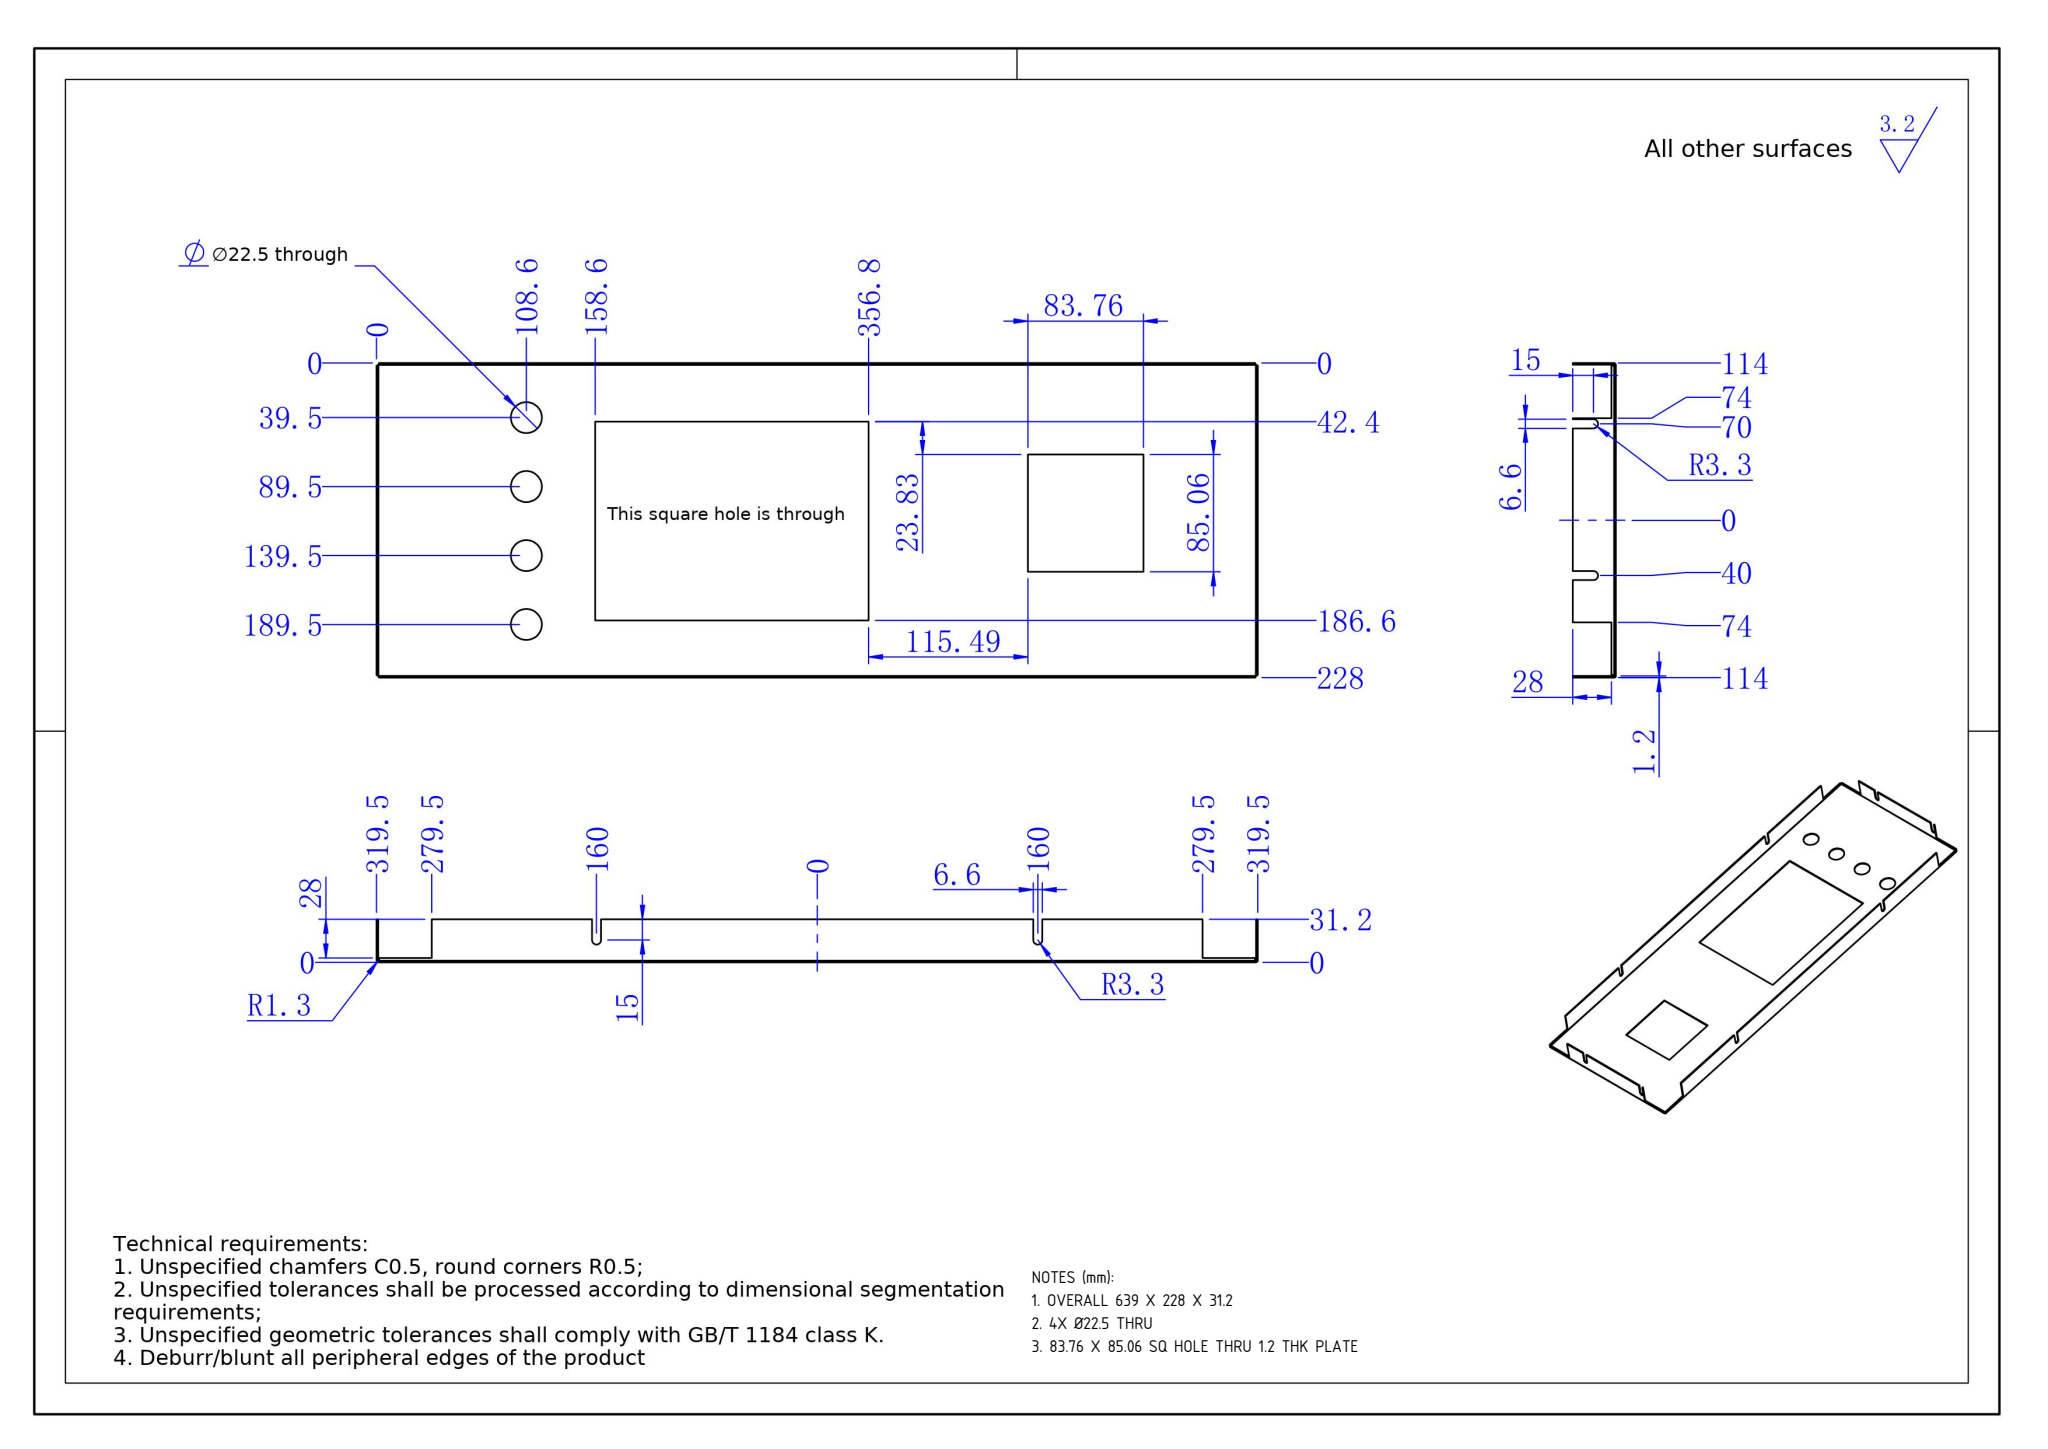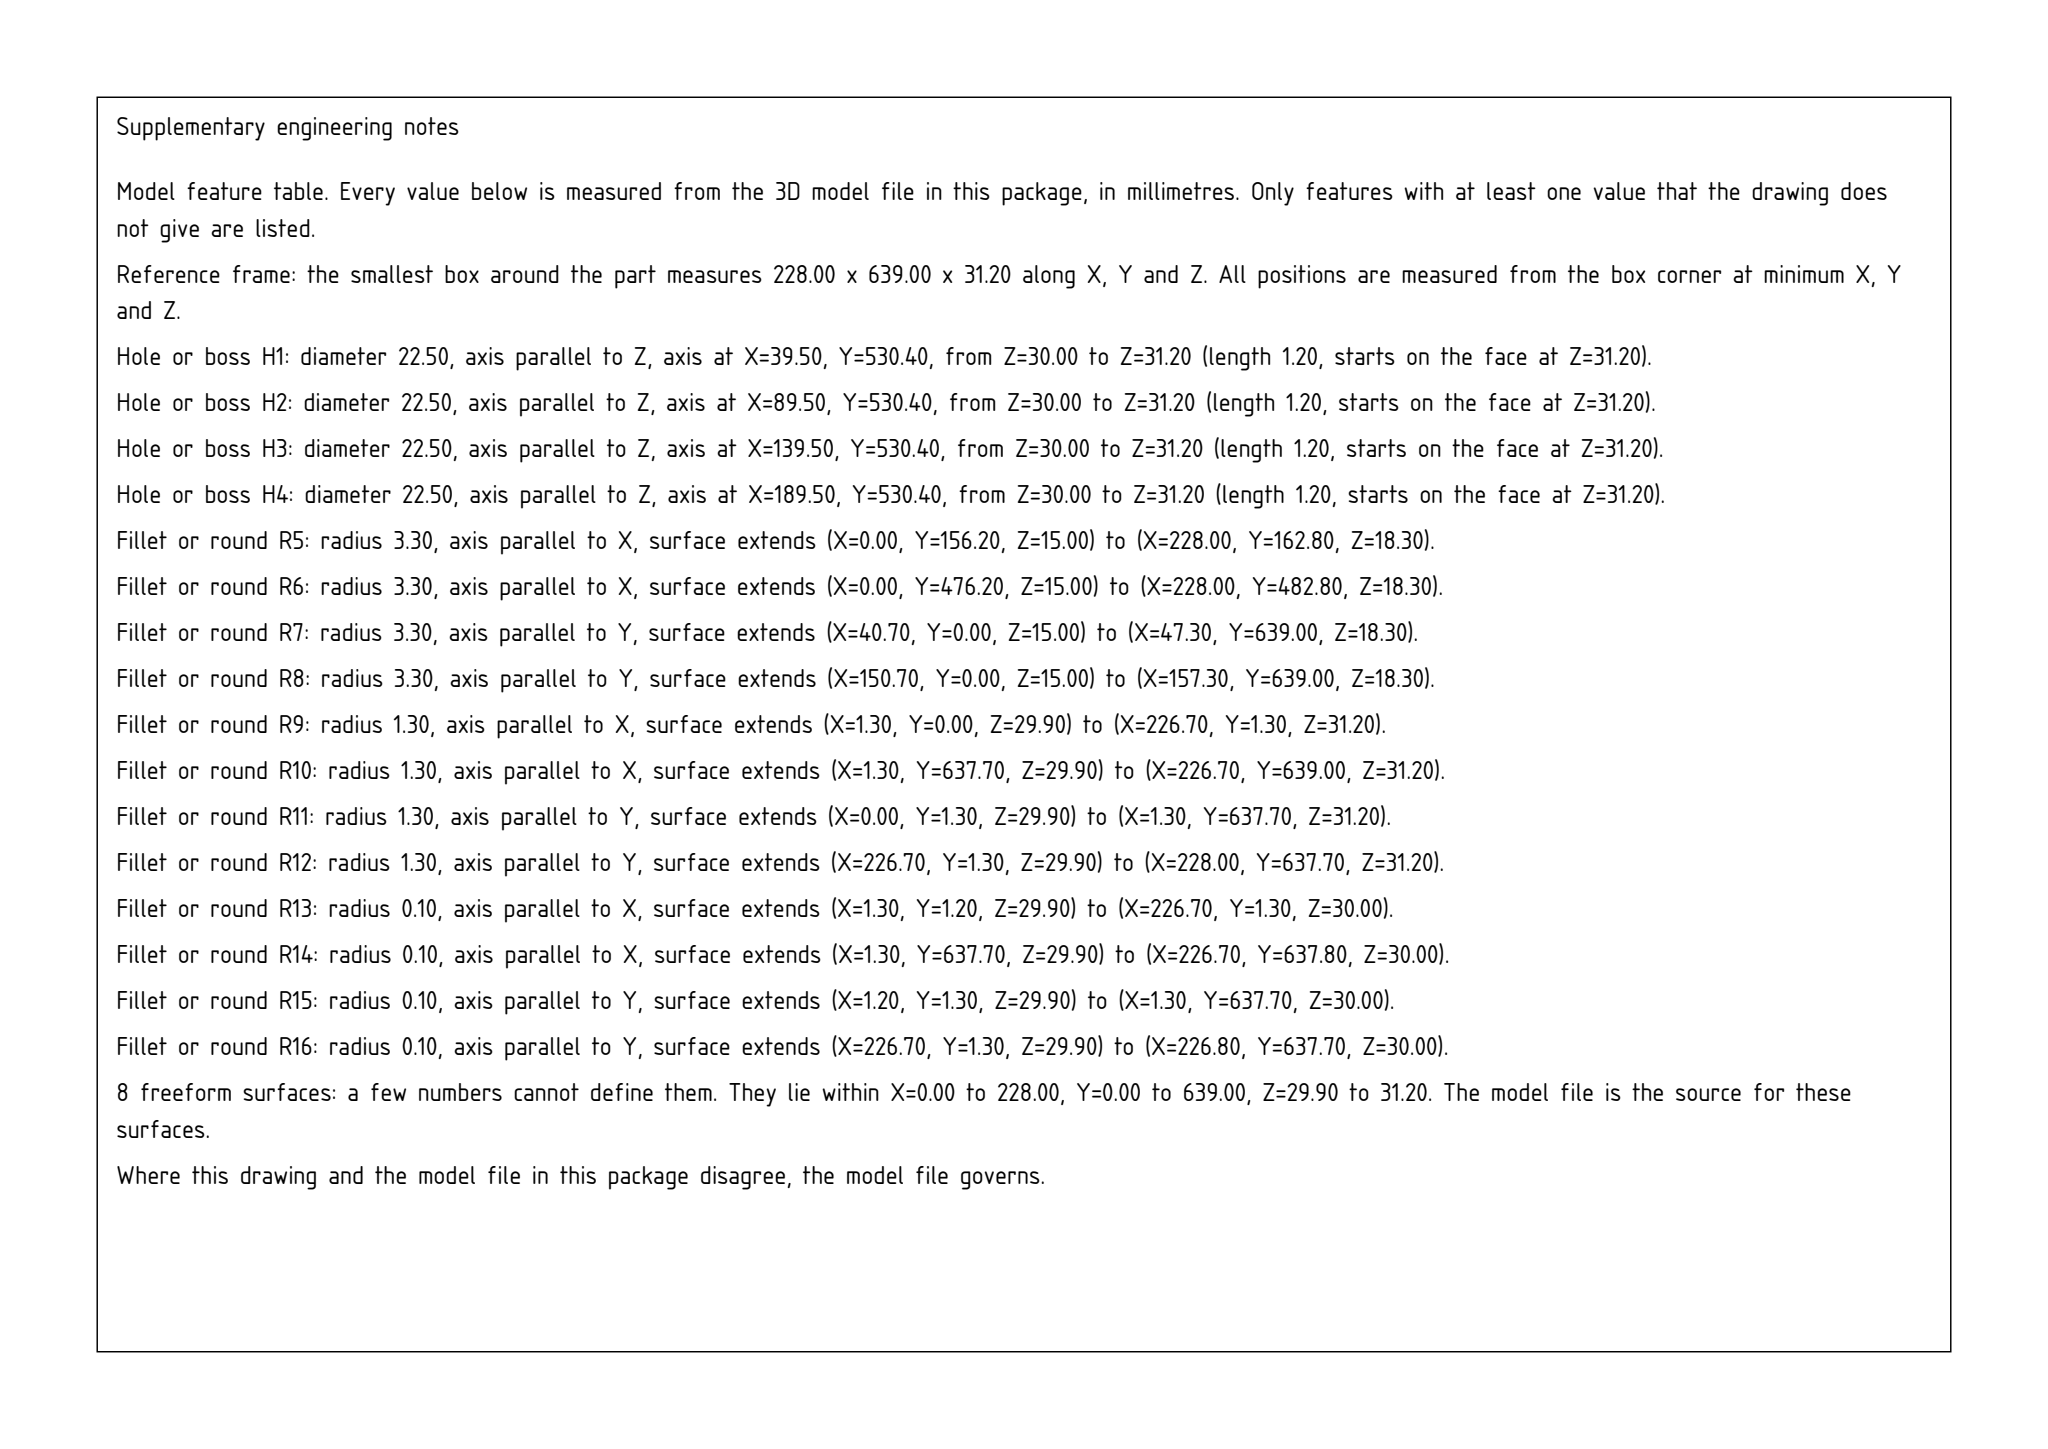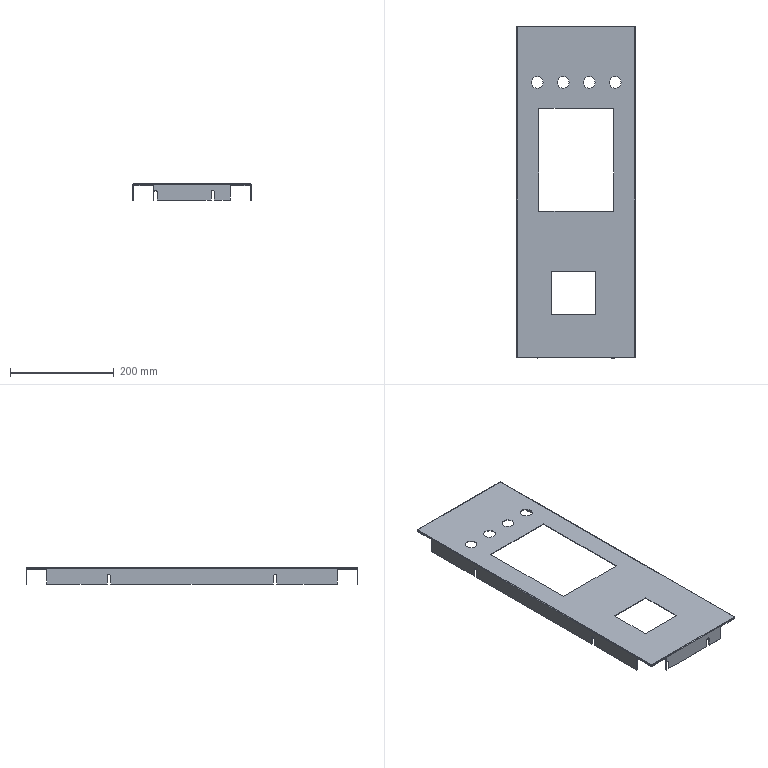Part | SolidWorks | mm | 1 solid | 106 faces | box 228 x 639 x 31.2 mm | volume 179964 mm3 | plane 70 | cylinder 28 | spline 8 | commonest cylinder face diameters 6.6 x12 22.5 x8 2.6 x4 0.2 x4
Drawing notes:
OVERALL 639 X 228 X 31.2 | from the solid: bbox_xyz 228.024 x 639.024 x 31.212
4X Ø22.5 THRU | from the solid: 4 cylinders Ø22.5 axis z, len 1.2 (= plate thk) at x=39.51/89.51/139.51/189.51, y=530.41
83.76 X 85.06 SQ HOLE THRU 1.2 THK PLATE | from the solid: Planes x66.25/151.31 (85.06) & y82.97/166.72 (83.75); plate z30.0-31.2 = 1.2 thk, no bottom face -> thru